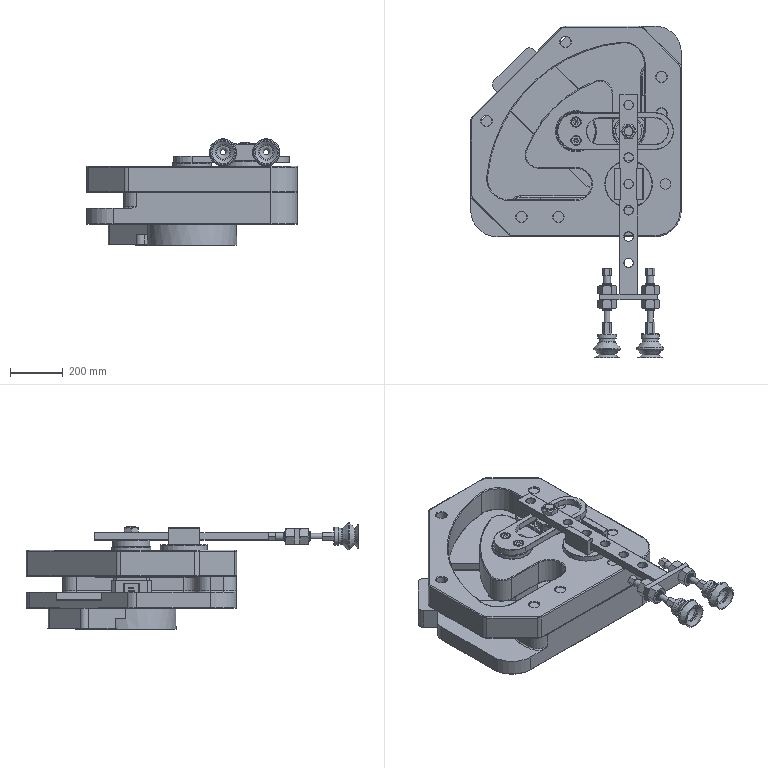Assembly | NX | mm | 28 component files | 29 solids | 1102 faces | box 800 x 1261.2 x 404.6 mm | volume 94011893 mm3 | plane 473 | cylinder 397 | torus 135 | cone 77 | sphere 16 | spline 4 | commonest cylinder face diameters 2 x149 8 x38 40 x26 12 x14 100 x13 23 x12 65 x12 1 x12
Bill of materials:
GB-T6170_F-2000,M39x4 | 4 |  | Tall hexagonal nut-like body with a central round through-bore and chamfered corners on both end faces.
unnamed part 1 | 4 |  | Solid stepped cylindrical pin: a short wide cylindrical base with a longer, narrower coaxial cylindrical shaft.
unnamed part 2 | 1 |  | Box-shaped body with chamfered vertical corners, a stepped top face, a raised circular boss and a protruding shaft with a flat; a rectangular block sticks out from one side.
unnamed part 3 | 1 |  | Thick flat plate with an irregular outline (chamfered corners and one rounded corner), a large curved slot cutout, an inner island area holding two large round holes, and many small holes around the edge.
unnamed part 4 | 1 |  | Coaxial stepped cylinder: a thin wide flange disc at the base, a large cylindrical body, a slightly smaller cylindrical step and a small cylindrical pin on top.
unnamed part 5 | 1 |  | Thin hexagonal nut-like body with a large central round through-bore and a chamfer on one end face.
unnamed part 6 | 1 |  | Flat circular washer-like ring with a central round hole.
unnamed part 7 | 2 |  | Screw-like part with a cylindrical head that has a hexagonal socket recess, and a plain cylindrical shank.
unnamed part 8 | 1 |  | Solid short cylinder with two small holes in one end face, placed symmetrically about the center.
unnamed part 9 | 1 |  | Corner plate with a large base slab, a raised L-shaped flange carrying a row of holes, and an angled rectangular tab sticking out diagonally; a rectangular block projects from the underside.
unnamed part 10 | 2 |  | Elongated axisymmetric part with a flared cup-shaped end, a collar, hex sections, a smooth stem, a ribbed/threaded section and a hex end.
unnamed part 11 | 1 |  | T-shaped flat bar: a long narrow strip with a row of seven round holes, joined at one end to a short perpendicular plate with two round holes.
unnamed part 12 | 1 |  | Short solid cylindrical body with a thin, slightly larger flange at its base. A rectangular block rises from the top face, and a straight channel runs through it with inward-facing lips at the top, giving a C-shaped (T-slot-like) undercut cross-section.
unnamed part 13 | 6 |  | Plain, solid-looking cylindrical pin with a short collar or head of larger diameter at one end. The shaft is much longer than the collar is tall.
unnamed part 14 | 1 |  | Flat plate shaped like a long rounded slot (obround), with fully rounded ends. A large obround cutout passes through most of its length, leaving a narrow rim. The solid end area has two small through-holes, each with a counterbore or countersink.
Mates:
1. touch align | A_Part_5 1 face | A_Part_6 1 face
2. touch align | A_Part_6 1 face | A_Part_5 1 face
3. touch align | Round_Hole_Washer 1 face | A_Part_6 1 face
4. touch align | Round_Hole_Washer 1 face | A_Part_6 1 face
5. touch align | A_Part_8 1 face | A_Part_5 1 face
6. touch align | A_Part_8 1 | A_Part_5 1 face
7. touch align | A_Part_2 1 face | A_Part_5 1 face
8. touch align | A_Part_2 1 face | A_Part_5 1 face
9. touch align | A_Part_1 1 face | A_Part_8 1 face
10. touch align | A_Part_1 1 face | A_Part_8 1 face
11. touch align | A_Part_1 1 face | A_Part_6 1 face
12. touch align | A_Part_1 1 face | A_Part_8 1 face
13. touch align | A_Hex_Screw 2 face | A_Part_8 1 face
14. touch align | A_Hex_Screw 1 face | A_Part_8 1 face
15. touch align | A_Hex_Screw 2 face | A_Part_1 1 face
16. touch align | A_Hex_Screw 1 face | A_Part_1 1 face
17. touch align | Transition_Actuator_Flange 1 face | A_Part_5 1 face
18. touch align | Transition_Actuator_Flange 1 face | A_Part_5 1 face
19. touch align | Transition_Actuator_Flange 1 face | A_Part_5 1 face
20. touch align | Transition_Actuator_Flange 1 face | A_Part_5 1 face
21. touch align | Transition_Actuator_Flange 1 face | A_Part_5 1 face
22. touch align | Transition_Actuator_Flange 1 face | A_Part_5 1 face
23. touch align | Transition_Actuator_Flange 1 face | A_Part_5 1 face
24. touch align | Transition_Actuator_Flange_Screw 3 face | A_Part_5 1 face
25. touch align | Transition_Actuator_Flange_Screw 3 face | Transition_Actuator_Flange 1 face
26. touch align | Transition_Actuator_Flange_Screw 4 face | Transition_Actuator_Flange 1 face
27. touch align | Transition_Actuator_Flange_Screw 4 face | Transition_Actuator_Flange 1 face
28. touch align | Transition_Actuator_Flange_Screw 6 face | Transition_Actuator_Flange 1 face
29. touch align | Transition_Actuator_Flange_Screw 6 face | Transition_Actuator_Flange 1 face
30. touch align | Transition_Actuator_Flange_Screw 5 face | Transition_Actuator_Flange 1 face
31. touch align | Transition_Actuator_Flange_Screw 5 face | Transition_Actuator_Flange 1 face
32. touch align | Transition_Actuator_Flange_Screw 2 face | Transition_Actuator_Flange 1 face
33. touch align | Transition_Actuator_Flange_Screw 1 face | Transition_Actuator_Flange 1 face
34. touch align | Transition_Actuator_Flange_Screw 2 face | Transition_Actuator_Flange 1 face
35. touch align | Transition_Actuator_Flange_Screw 1 face | Transition_Actuator_Flange 1 face
36. touch align | assembly face | Transition_Actuator_Flange 1 face
37. touch align | A_Part_8 1 | assembly face
38. touch align | A_Part_3 1 face | A_Part_6 1 face
39. touch align | A_Part_3 1 face | Round_Hole_Washer 1 face
40. touch align | A_Suction_Cup 2 face | A_Part_3 1 face
41. touch align | A_Suction_Cup 1 face | A_Part_3 1 face
42. touch align | GB-T6170_F-2000_M39x4 4 face | A_Suction_Cup 2 face
43. touch align | GB-T6170_F-2000_M39x4 3 face | A_Suction_Cup 1 face
44. touch align | GB-T6170_F-2000_M39x4 4 face | A_Part_3 1 face
45. touch align | GB-T6170_F-2000_M39x4 3 face | A_Part_3 1 face
46. touch align | GB-T6170_F-2000_M39x4 2 face | A_Suction_Cup 2 face
47. touch align | GB-T6170_F-2000_M39x4 1 face | A_Suction_Cup 1 face
48. touch align | GB-T6170_F-2000_M39x4 1 face | A_Part_3 1 face
49. touch align | GB-T6170_F-2000_M39x4 2 face | A_Part_3 1 face
50. touch align | A_Part_10 1 face | A_Part_6 1 face
51. touch align | A_Part_10 1 face | A_Part_3 1 face
52. touch align | Flange_Transition_Bolt 1 face | Transition_Actuator_Flange 1 face
53. touch align | Flange_Transition_Bolt 2 face | Transition_Actuator_Flange 1 face
54. touch align | Flange_Transition_Bolt 3 face | Transition_Actuator_Flange 1 face
55. touch align | Flange_Transition_Bolt 4 face | Transition_Actuator_Flange 1 face
56. touch align | Flange_Transition_Bolt 4 face | Transition_Actuator_Flange 1 face
57. touch align | Flange_Transition_Bolt 1 face | Transition_Actuator_Flange 1 face
58. touch align | Flange_Transition_Bolt 2 face | Transition_Actuator_Flange 1 face
59. touch align | Flange_Transition_Bolt 3 face | Transition_Actuator_Flange 1 face
60. touch align | Integrated_Stepper_Motor 1 face | Transition_Actuator_Flange 1 face